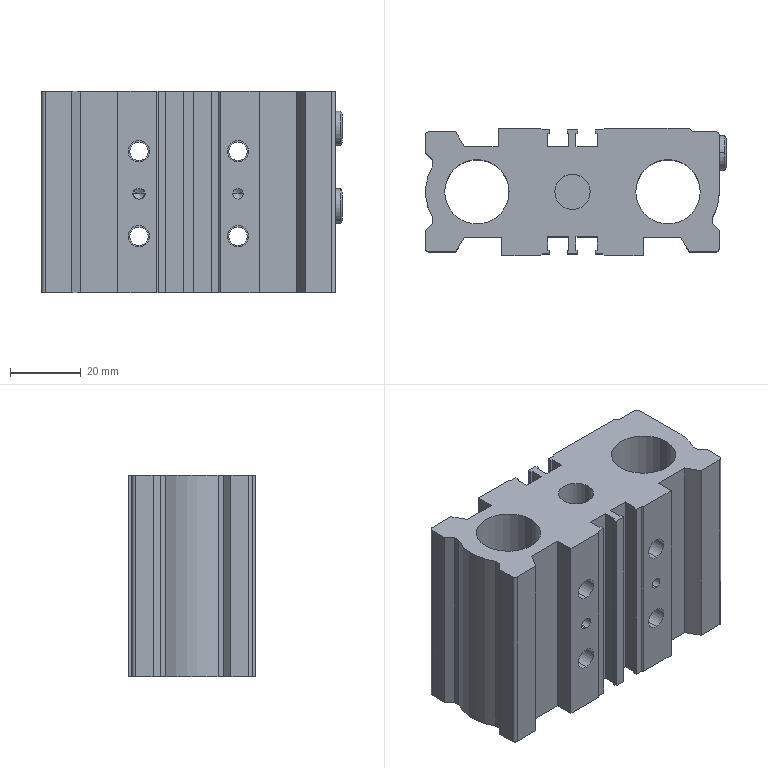Component | SolidWorks | 1-VASP2004STG-M-20-20-T0H-D-1_1-VASP2004STG-Body_A_default-1 | 1 solid | 229 faces | volume 98920 mm3 | plane 117 | cylinder 88 | cone 24 | commonest cylinder face diameters 3 x13 6 x8 9.5 x8 5 x8 5.2 x8 4.3 x8 18.2 x4 9.73 x4